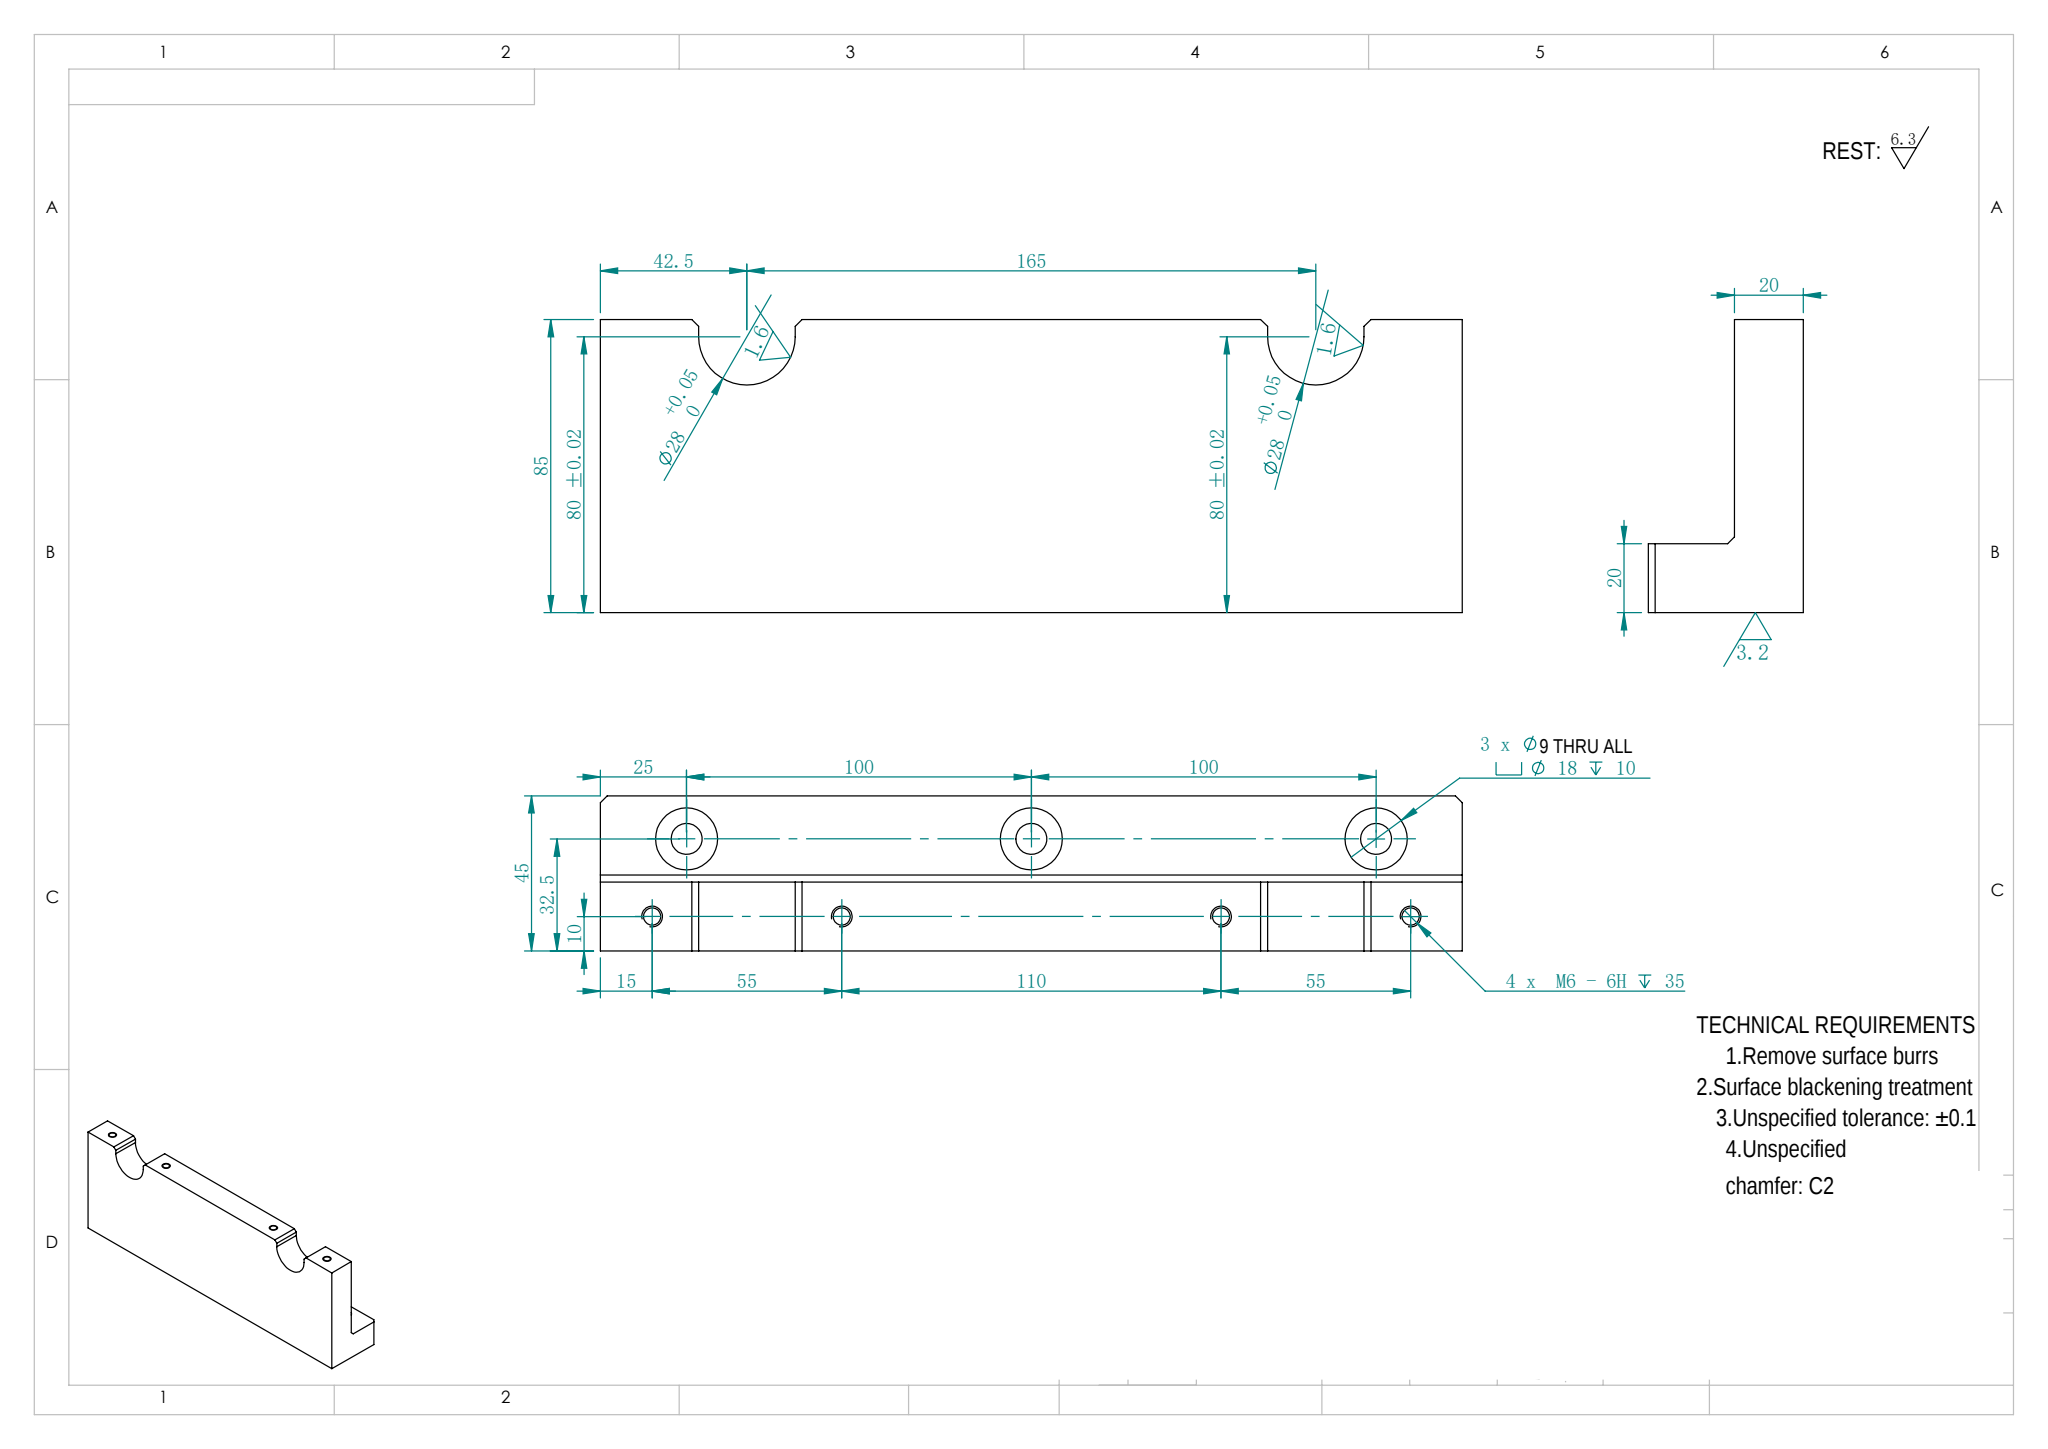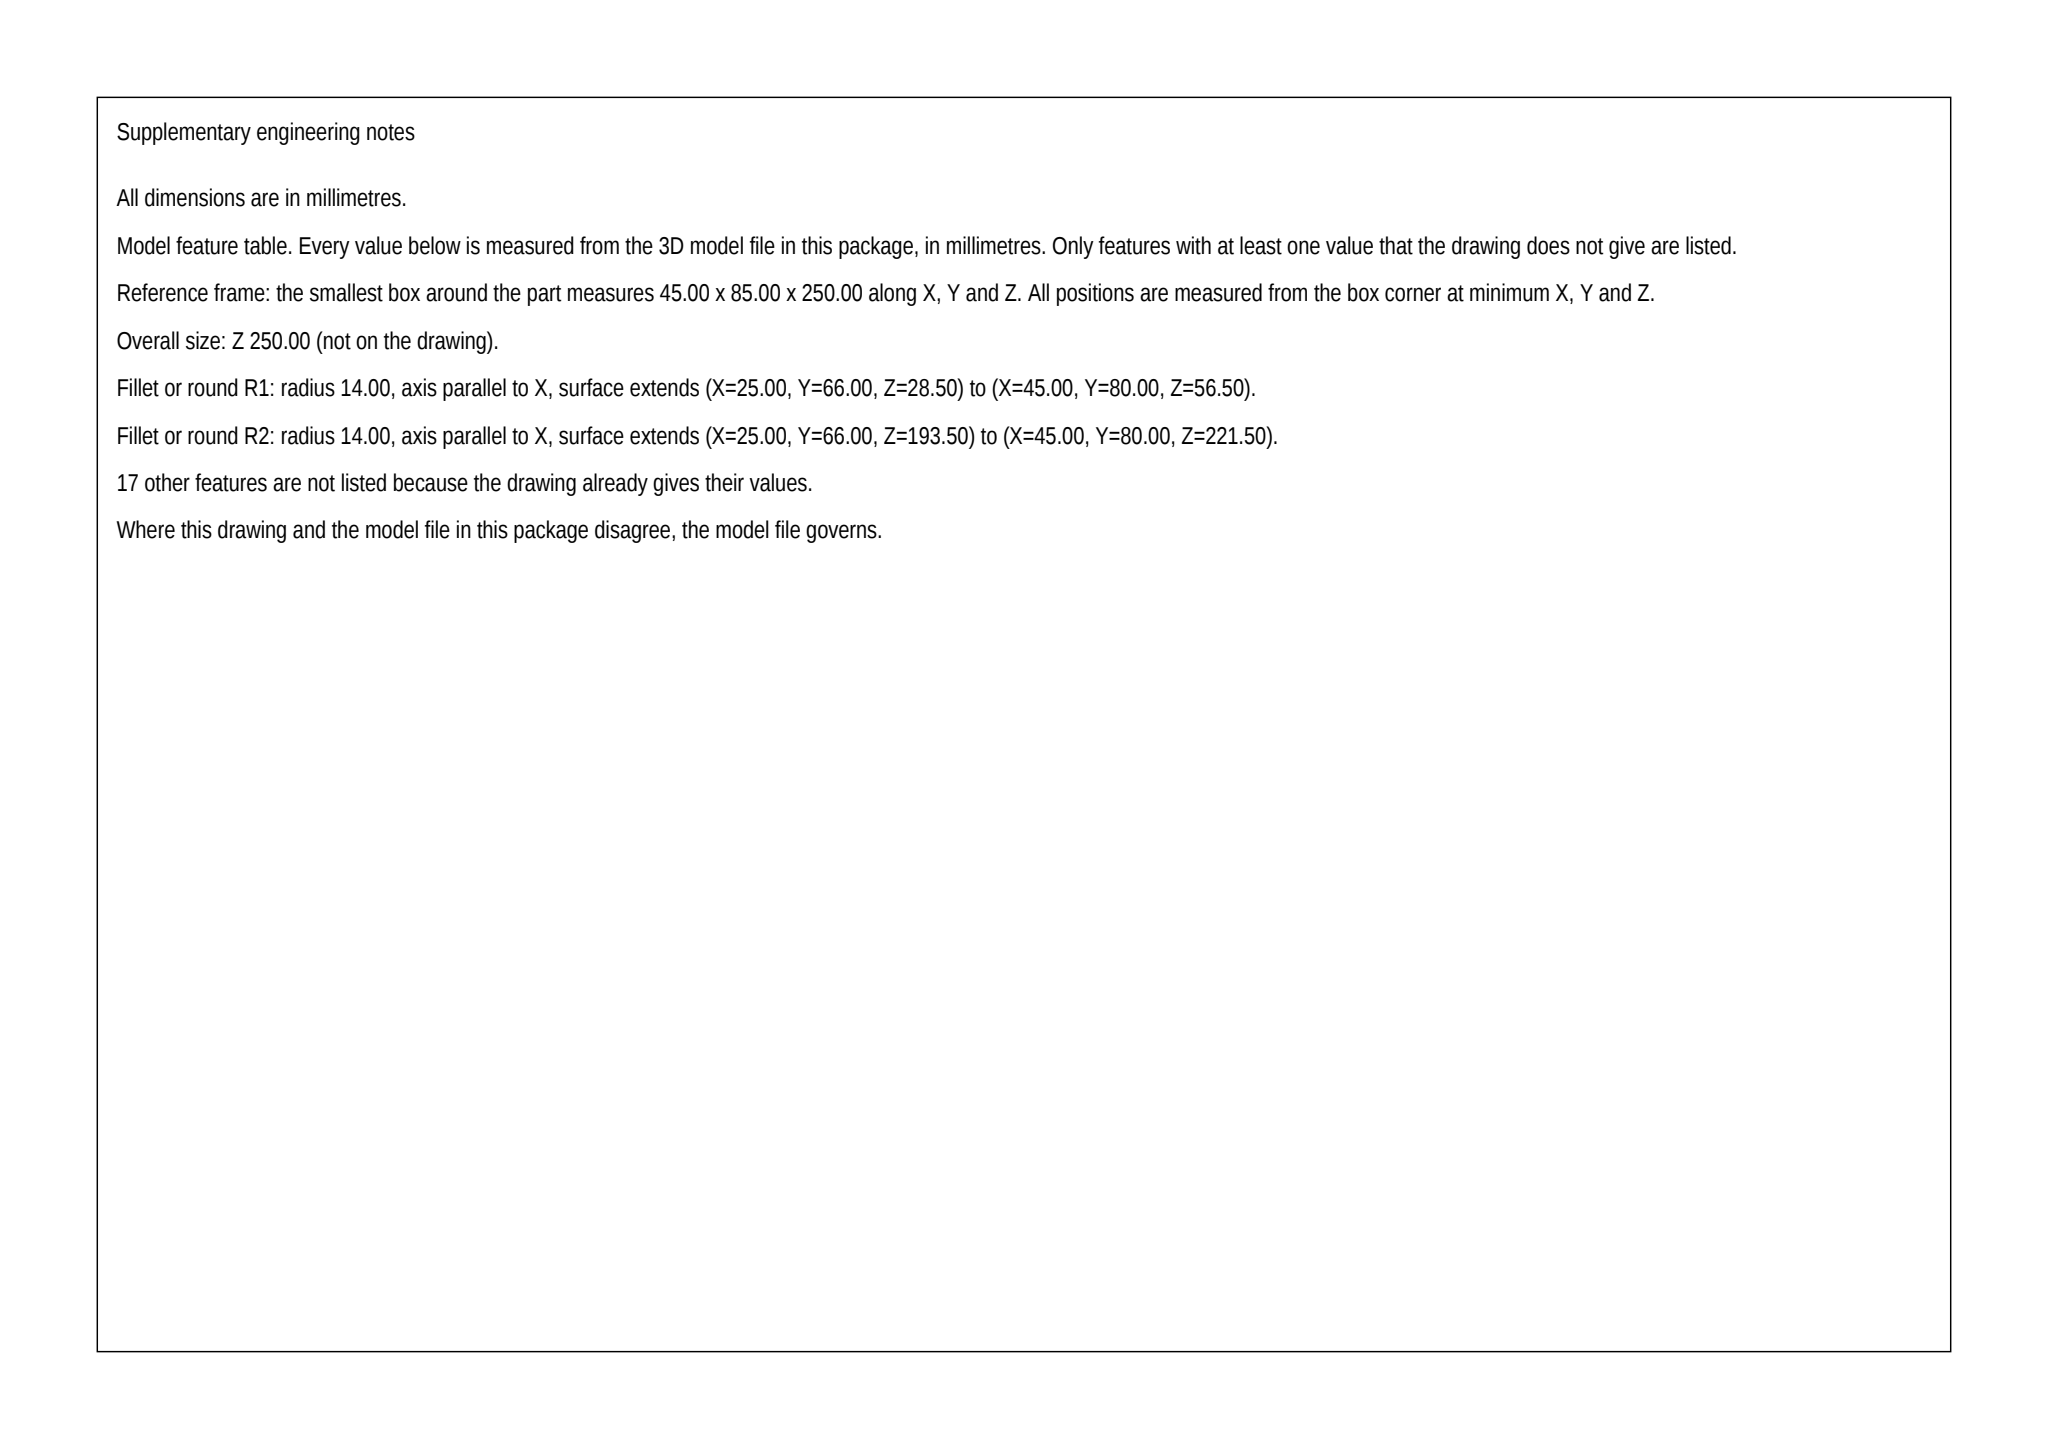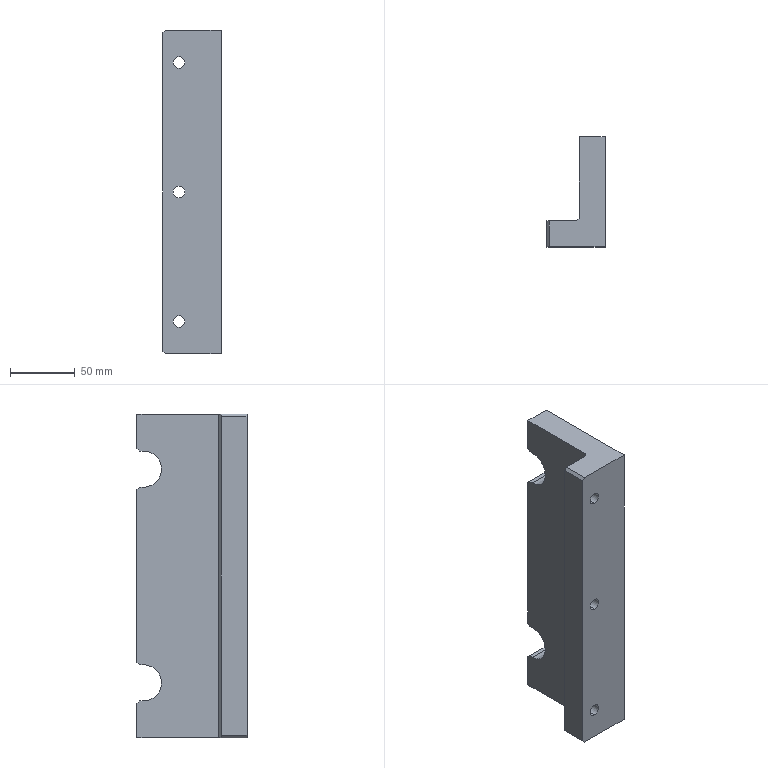Part | SolidWorks | mm | 1 solid | 54 faces | box 45 x 85 x 250 mm | volume 520014 mm3 | plane 24 | cylinder 22 | cone 8 | commonest cylinder face diameters 5 x8 18 x6 9 x6 28 x2
build123d program:
from build123d import *

# Parameters (mm, degrees)
BOSS_EXTRUDE1_DEPTH                                 = 250
CUT_EXTRUDE1_DEPTH                                  = 268.862
CYLINDRICAL_COUNTERSUNK_HOLE_FOR_M8_HEX_D           = 9
CYLINDRICAL_COUNTERSUNK_HOLE_FOR_M8_HEX_CBORE_D     = 18
CYLINDRICAL_COUNTERSUNK_HOLE_FOR_M8_HEX_CBORE_DEPTH = 10
M6_TAPPED_HOLE1_D                                   = 5
M6_TAPPED_HOLE1_DEPTH                               = 35
M6_TAPPED_HOLE1_TIP                                 = 1.502
CHAMFER1_SIZE                                       = 2


with BuildPart() as part:
    # Sketch1 → Boss-Extrude1 (new body)
    with BuildSketch(Plane.XY):
        Polygon((0, 85), (0, 0), (-45, 0), (-45, 20), (-20, 20), (-20, 85), align=None)
    extrude(amount=BOSS_EXTRUDE1_DEPTH)

    # Sketch2 → Cut-Extrude1 (cut, through all)
    with BuildSketch(Plane(origin=(0, 0, 0), x_dir=(0, 0, -1), z_dir=(1, 0, 0))):
        with BuildLine():
            Line((-221.5, 80), (-221.5, 100))
            ThreePointArc((-221.5, 100), (-207.5, 114), (-193.5, 100))
            Line((-193.5, 100), (-193.5, 80))
            ThreePointArc((-193.5, 80), (-207.5, 66), (-221.5, 80))
        make_face()
        with BuildLine():
            Line((-56.5, 80), (-56.5, 100))
            ThreePointArc((-56.5, 100), (-42.5, 114), (-28.5, 100))
            Line((-28.5, 100), (-28.5, 80))
            ThreePointArc((-28.5, 80), (-42.5, 66), (-56.5, 80))
        make_face()
    extrude(amount=-CUT_EXTRUDE1_DEPTH, mode=Mode.SUBTRACT)

    # Cylindrical Countersunk Hole for M8 Hex (through all)
    with Locations(Plane(origin=(0, 20, 0), x_dir=(1, 0, 0), z_dir=(0, 1, 0))):
        with Locations((-32.5, -225), (-32.5, -125), (-32.5, -25)):
            CounterBoreHole(CYLINDRICAL_COUNTERSUNK_HOLE_FOR_M8_HEX_D / 2, CYLINDRICAL_COUNTERSUNK_HOLE_FOR_M8_HEX_CBORE_D / 2, CYLINDRICAL_COUNTERSUNK_HOLE_FOR_M8_HEX_CBORE_DEPTH)

    # M6 Tapped Hole1
    with Locations(Plane(origin=(0, 85, 0), x_dir=(1, 0, 0), z_dir=(0, 1, 0))):
        with Locations((-10, -235), (-10, -180), (-10, -70), (-10, -15)):
            Hole(M6_TAPPED_HOLE1_D / 2, depth=M6_TAPPED_HOLE1_DEPTH)
            with Locations((0, 0, -(M6_TAPPED_HOLE1_DEPTH + M6_TAPPED_HOLE1_TIP / 2))):  # 118° drill point
                Cone(0, M6_TAPPED_HOLE1_D / 2, M6_TAPPED_HOLE1_TIP, mode=Mode.SUBTRACT)

    # Chamfer1
    chamfer1_edges = [part.edges().sort_by_distance(p)[0] for p in [
        (-20, 20, 125),
        (-45, 10, 250),
        (-10, 85, 221.5),
        (-10, 85, 193.5),
        (-10, 85, 56.5),
        (-10, 85, 28.5),
        (-45, 10, 0),
    ]]
    chamfer(chamfer1_edges, length=CHAMFER1_SIZE)


solid = part.part